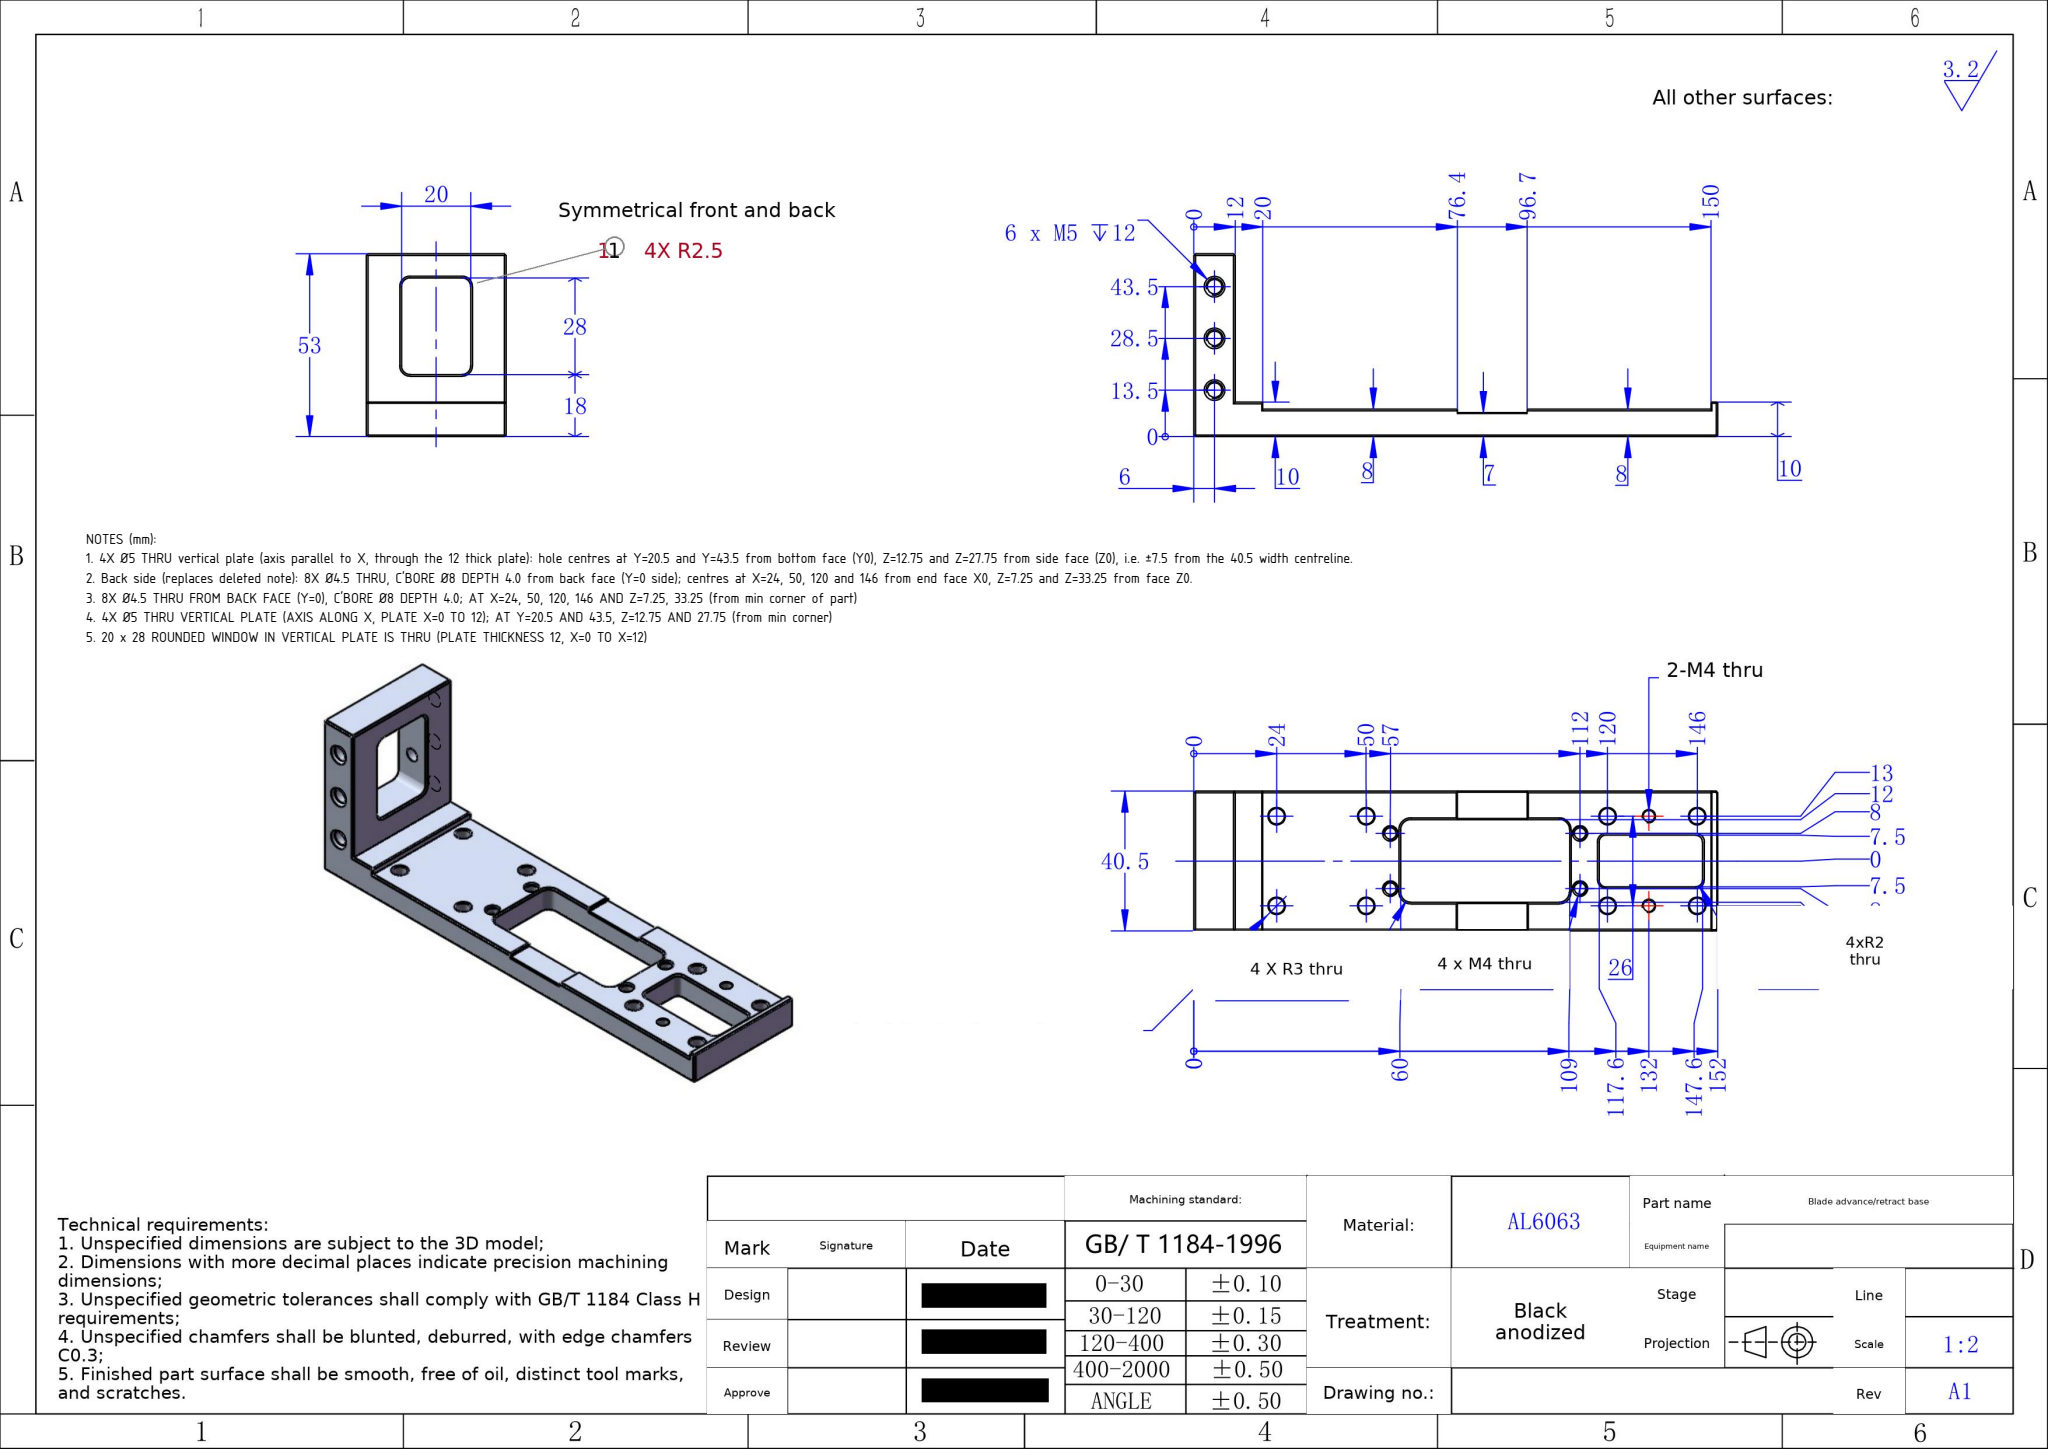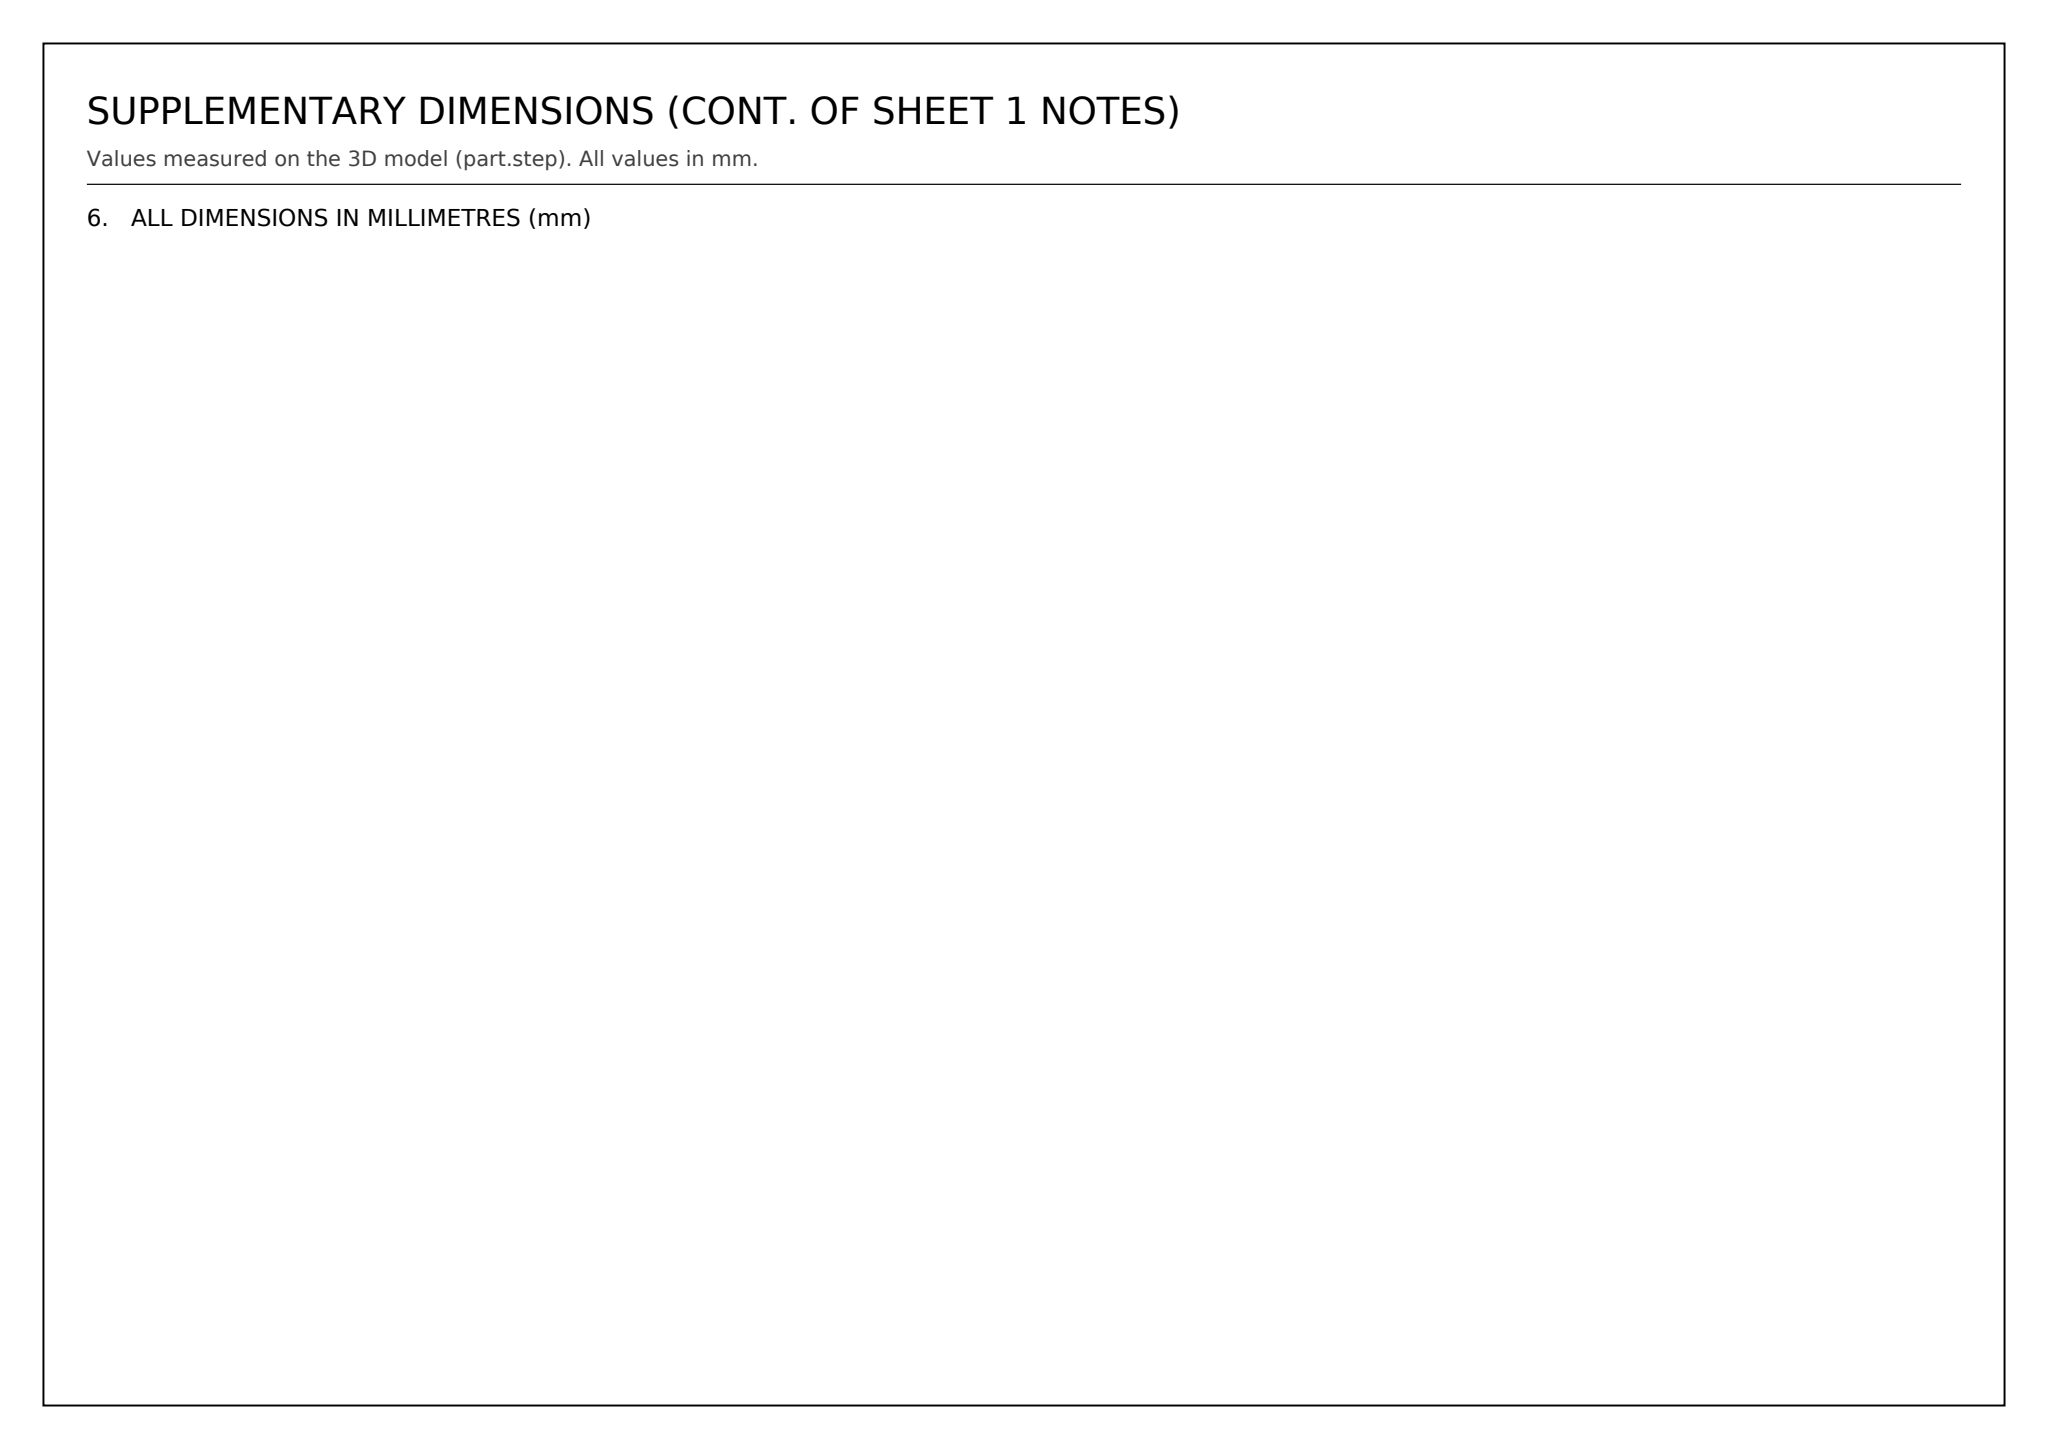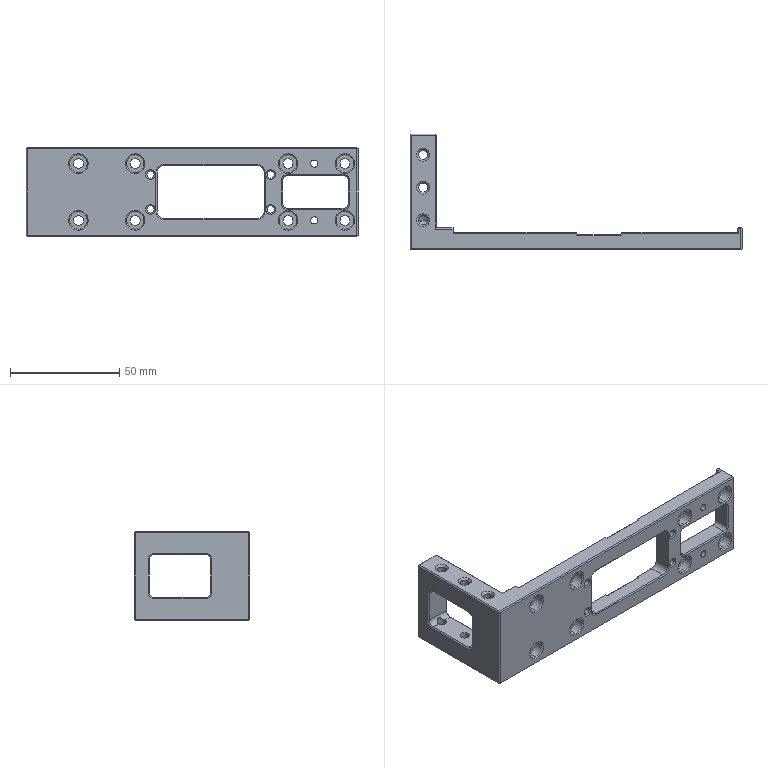Part | SolidWorks | mm | 1 solid | 262 faces | box 152 x 53 x 40.5 mm | volume 48083 mm3 | plane 106 | cone 88 | cylinder 68 | commonest cylinder face diameters 8 x16 4.5 x16 3.3 x12 4.2 x12 6 x4 4 x4 5 x4
Drawing notes:
4X Ø5 THRU vertical plate (axis parallel to X, through the 12 thick plate): hole centres at Y=20.5 and Y=43.5 from bottom face (Y0), Z=12.75 and Z=27.75 from side face (Z0), i.e. ±7.5 from the 40.5 width centreline. | from the solid: cylinders [5.0,"x",[null,20.5,12.75],11.0], [5.0,"x",[null,20.5,27.75],11.0], [5.0,"x",[null,43.5,12.75],11.0], [5.0,"x",[null,43.5,27.75],11.0]
Back side (replaces deleted note): 8X Ø4.5 THRU, C'BORE Ø8 DEPTH 4.0 from back face (Y=0 side); centres at X=24, 50, 120 and 146 from end face X0, Z=7.25 and Z=33.25 from face Z0. | from the solid: cylinders [4.5,"y",[24.0/50.0/120.0/146.0,null,7.25 & 33.25],3.2] with coaxial [8.0,"y",same positions,4.0]
8X Ø4.5 THRU FROM BACK FACE (Y=0), C'BORE Ø8 DEPTH 4.0; AT X=24, 50, 120, 146 AND Z=7.25, 33.25 (from min corner of part) | from the solid: cylinders [4.5,'y',[24/50/120/146,null,7.25 & 33.25],3.2] with coaxial [8.0,'y',same,4.0]
4X Ø5 THRU VERTICAL PLATE (AXIS ALONG X, PLATE X=0 TO 12); AT Y=20.5 AND 43.5, Z=12.75 AND 27.75 (from min corner) | from the solid: cylinders [5.0,'x',[null,20.5/43.5,12.75/27.75],11.0] ×4
20 x 28 ROUNDED WINDOW IN VERTICAL PLATE IS THRU (PLATE THICKNESS 12, X=0 TO X=12) | from the solid: axis_planes x=0.0 and x=12.0 are the two vertical-plate faces; no intermediate floor plane between them
ALL DIMENSIONS IN MILLIMETRES (mm) | from the solid: STEP model units mm, bbox_xyz [152.0, 53.0, 40.5]